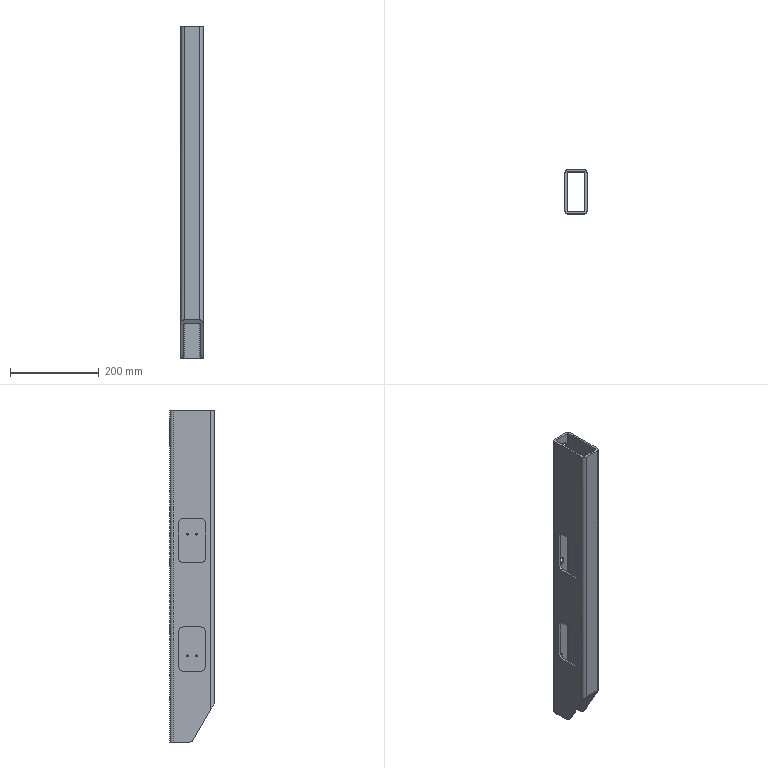Component | SolidWorks | JHK-B1002RightRectangularTubeBeam-1 | 1 solid | 79 faces | box 50 x 100 x 750 mm | volume 904420 mm3 | cylinder 52 | plane 27 | commonest cylinder face diameters 20 x14 3.3 x12 4.2 x8 12 x6 30 x4 15 x4 5 x4 | material Q235A
build123d program:
from build123d import *

# Parameters (mm, degrees)
EXTRUDE_THIN1_DEPTH   = 375
CUT_EXTRUDE1_REACH    = 383.608
CUT_EXTRUDE2_REACH    = 383.608
SKETCH5_R             = 15
CUT_EXTRUDE3_DEPTH    = 382.608
CUT_EXTRUDE4_REACH    = 390.909
M4_TAPPED_HOLE2_D     = 3.3
M4_TAPPED_HOLE2_DEPTH = 5
M5_TAPPED_HOLE1_D     = 4.2
M5_TAPPED_HOLE1_DEPTH = 5
FILLET1_R             = 10
CUT_EXTRUDE5_REACH    = 390.909


with BuildPart() as part:
    # Sketch1 → Extrude-Thin1 (new, symmetric)
    with BuildSketch(Plane.XY):
        with BuildLine():
            Line((17.5, 50), (-17.5, 50))
            ThreePointArc((-17.5, 50), (-22.803, 47.803), (-25, 42.5))
            Line((-25, 42.5), (-25, -42.5))
            ThreePointArc((-25, -42.5), (-22.803, -47.803), (-17.5, -50))
            Line((-17.5, -50), (17.5, -50))
            ThreePointArc((17.5, -50), (22.803, -47.803), (25, -42.5))
            Line((25, -42.5), (25, 42.5))
            ThreePointArc((25, 42.5), (22.803, 47.803), (17.5, 50))
        make_face()
        with BuildLine():
            Line((17.5, 45), (-17.5, 45))
            ThreePointArc((-17.5, 45), (-19.268, 44.268), (-20, 42.5))
            Line((-20, 42.5), (-20, -42.5))
            ThreePointArc((-20, -42.5), (-19.268, -44.268), (-17.5, -45))
            Line((-17.5, -45), (17.5, -45))
            ThreePointArc((17.5, -45), (19.268, -44.268), (20, -42.5))
            Line((20, -42.5), (20, 42.5))
            ThreePointArc((20, 42.5), (19.268, 44.268), (17.5, 45))
        make_face(mode=Mode.SUBTRACT)
    extrude(amount=EXTRUDE_THIN1_DEPTH, both=True)

    # Sketch2 → Cut-Extrude1 (cut, up to next)
    with BuildSketch(Plane.ZY.offset(25), mode=Mode.PRIVATE) as cut_extrude1_sk1:
        with BuildLine():
            Line((40, -30), (120, -30))
            ThreePointArc((120, -30), (127.071, -27.071), (130, -20))
            Line((130, -20), (130, 20))
            ThreePointArc((130, 20), (127.071, 27.071), (120, 30))
            Line((120, 30), (40, 30))
            ThreePointArc((40, 30), (32.929, 27.071), (30, 20))
            Line((30, 20), (30, -20))
            ThreePointArc((30, -20), (32.929, -27.071), (40, -30))
        make_face()
    cut_extrude1_tool1 = extrude(cut_extrude1_sk1.sketch, amount=-CUT_EXTRUDE1_REACH, mode=Mode.PRIVATE) & part.part
    # Sketch2 → Cut-Extrude1 (cut, up to next)
    with BuildSketch(Plane.ZY.offset(25), mode=Mode.PRIVATE) as cut_extrude1_sk2:
        with BuildLine():
            Line((-215, -20), (-215, 20))
            ThreePointArc((-215, 20), (-212.071, 27.071), (-205, 30))
            Line((-205, 30), (-125, 30))
            ThreePointArc((-125, 30), (-117.929, 27.071), (-115, 20))
            Line((-115, 20), (-115, -20))
            ThreePointArc((-115, -20), (-117.929, -27.071), (-125, -30))
            Line((-125, -30), (-205, -30))
            ThreePointArc((-205, -30), (-212.071, -27.071), (-215, -20))
        make_face()
    cut_extrude1_tool2 = extrude(cut_extrude1_sk2.sketch, amount=-CUT_EXTRUDE1_REACH, mode=Mode.PRIVATE) & part.part
    add(cut_extrude1_tool1.solids().sort_by_distance((-25, 0, 80))[0], mode=Mode.SUBTRACT)
    add(cut_extrude1_tool2.solids().sort_by_distance((-25, 0, -165))[0], mode=Mode.SUBTRACT)

    # Sketch5 → Cut-Extrude2 (cut, up to next)
    with BuildSketch(Plane(origin=(25, 0, 0), x_dir=(0, 0, -1), z_dir=(1, 0, 0)), mode=Mode.PRIVATE) as cut_extrude2_sk1:
        with Locations((-175, 0)):
            Circle(SKETCH5_R)
    cut_extrude2_tool1 = extrude(cut_extrude2_sk1.sketch, amount=-CUT_EXTRUDE2_REACH, mode=Mode.PRIVATE) & part.part
    # Sketch5 → Cut-Extrude2 (cut, up to next)
    with BuildSketch(Plane(origin=(25, 0, 0), x_dir=(0, 0, -1), z_dir=(1, 0, 0)), mode=Mode.PRIVATE) as cut_extrude2_sk2:
        with Locations((245, 0)):
            Circle(SKETCH5_R)
    cut_extrude2_tool2 = extrude(cut_extrude2_sk2.sketch, amount=-CUT_EXTRUDE2_REACH, mode=Mode.PRIVATE) & part.part
    add(cut_extrude2_tool1.solids().sort_by_distance((25, 0, 175))[0], mode=Mode.SUBTRACT)
    add(cut_extrude2_tool2.solids().sort_by_distance((25, 0, -245))[0], mode=Mode.SUBTRACT)

    # Sketch6 → Cut-Extrude3 (cut, through all)
    with BuildSketch(Plane(origin=(25, 0, 0), x_dir=(0, 0, -1), z_dir=(1, 0, 0))):
        Polygon((375, 0), (288.397, -50), (375, -50), align=None)
    extrude(amount=-CUT_EXTRUDE3_DEPTH, mode=Mode.SUBTRACT)

    # Sketch7 → Cut-Extrude4 (cut, up to next)
    with BuildSketch(Plane(origin=(0, 50, 0), x_dir=(1, 0, 0), z_dir=(0, 1, 0)), mode=Mode.PRIVATE) as cut_extrude4_sk1:
        with BuildLine():
            Line((-5, -355), (5, -355))
            ThreePointArc((5, -355), (12.071, -352.071), (15, -345))
            Line((15, -345), (15, -305))
            ThreePointArc((15, -305), (12.071, -297.929), (5, -295))
            Line((5, -295), (-5, -295))
            ThreePointArc((-5, -295), (-12.071, -297.929), (-15, -305))
            Line((-15, -305), (-15, -345))
            ThreePointArc((-15, -345), (-12.071, -352.071), (-5, -355))
        make_face()
    cut_extrude4_tool1 = extrude(cut_extrude4_sk1.sketch, amount=-CUT_EXTRUDE4_REACH, mode=Mode.PRIVATE) & part.part
    add(cut_extrude4_tool1.solids().sort_by_distance((0, 50, 325))[0], mode=Mode.SUBTRACT)

    # M4 Tapped Hole2
    with Locations(Plane(origin=(25, 1.867, 74.937), x_dir=(0, 0, -1), z_dir=(1, 0, 0))):
        with Locations((-19.063, 8.133), (254.937, 8.133), (-19.063, -11.867), (254.937, -11.867), (349.711, 18.646), (368.937, 13.133)):
            Hole(M4_TAPPED_HOLE2_D / 2, depth=M4_TAPPED_HOLE2_DEPTH)

    # M5 Tapped Hole1
    with Locations(Plane(origin=(0, 50, 0), x_dir=(1, 0, 0), z_dir=(0, 1, 0))):
        with Locations((0, 226), (0, 276), (0, -190), (0, -140)):
            Hole(M5_TAPPED_HOLE1_D / 2, depth=M5_TAPPED_HOLE1_DEPTH)

    # Fillet1
    fillet1_edges = [part.edges().sort_by_distance(p)[0] for p in [
        (-22.5, 0, -375),
        (22.5, 0, -375),
    ]]
    fillet(fillet1_edges, radius=FILLET1_R)

    # Sketch12 → Cut-Extrude5 (cut, up to next)
    with BuildSketch(Plane(origin=(0, 50, 0), x_dir=(1, 0, 0), z_dir=(0, 1, 0)), mode=Mode.PRIVATE) as cut_extrude5_sk1:
        with BuildLine():
            Line((6, 120.5), (6, 115.5))
            ThreePointArc((6, 115.5), (0, 109.5), (-6, 115.5))
            Line((-6, 115.5), (-6, 120.5))
            ThreePointArc((-6, 120.5), (0, 126.5), (6, 120.5))
        make_face()
    cut_extrude5_tool1 = extrude(cut_extrude5_sk1.sketch, amount=-CUT_EXTRUDE5_REACH, mode=Mode.PRIVATE) & part.part
    # Sketch12 → Cut-Extrude5 (cut, up to next)
    with BuildSketch(Plane(origin=(0, 50, 0), x_dir=(1, 0, 0), z_dir=(0, 1, 0)), mode=Mode.PRIVATE) as cut_extrude5_sk2:
        with BuildLine():
            Line((6, -29.5), (6, -34.5))
            ThreePointArc((6, -34.5), (0, -40.5), (-6, -34.5))
            Line((-6, -34.5), (-6, -29.5))
            ThreePointArc((-6, -29.5), (0, -23.5), (6, -29.5))
        make_face()
    cut_extrude5_tool2 = extrude(cut_extrude5_sk2.sketch, amount=-CUT_EXTRUDE5_REACH, mode=Mode.PRIVATE) & part.part
    add(cut_extrude5_tool1.solids().sort_by_distance((0, 50, -118))[0], mode=Mode.SUBTRACT)
    add(cut_extrude5_tool2.solids().sort_by_distance((0, 50, 32))[0], mode=Mode.SUBTRACT)


solid = part.part

# Placed as in the assembly
solid = solid.moved(Location((295, -150, -520), (0, 0, 0)))